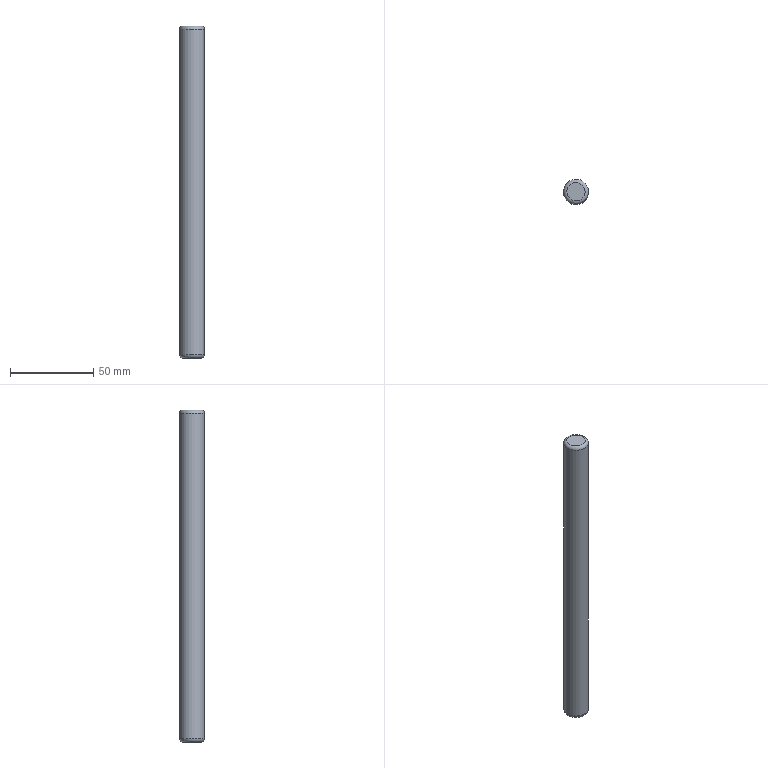Component | NX | CBK2 | 1 solid | 5 faces | box 15 x 15 x 200 mm | volume 35267 mm3 | plane 2 | torus 2 | cylinder 1 | commonest cylinder face diameters 15 x1
STEP:
#1=CARTESIAN_POINT('',(0.,0.,0.));
#2=DIRECTION('',(0.,0.,1.));
#3=DIRECTION('',(1.,0.,0.));
#4=AXIS2_PLACEMENT_3D('',#1,#2,#3);
#5=CARTESIAN_POINT('',(-1117.64,953.261,23.928));
#6=VERTEX_POINT('',#5);
#7=CARTESIAN_POINT('',(-1123.378,958.091,23.928));
#8=DIRECTION('',(0.,0.,1.));
#9=DIRECTION('',(0.7651,-0.644,0.));
#10=AXIS2_PLACEMENT_3D('',#7,#8,#9);
#11=CIRCLE('',#10,7.5);
#12=CARTESIAN_POINT('',(-1123.378,958.091,221.928));
#13=DIRECTION('',(0.,0.,-1.));
#14=DIRECTION('',(-0.7651,0.644,0.));
#15=AXIS2_PLACEMENT_3D('',#12,#13,#14);
#16=CYLINDRICAL_SURFACE('',#15,7.5);
#17=CARTESIAN_POINT('',(9.425,198.));
#18=DIRECTION('',(-1.,0.));
#19=VECTOR('',#18,1.);
#20=LINE('',#17,#19);
#21=(GEOMETRIC_REPRESENTATION_CONTEXT(2)PARAMETRIC_REPRESENTATION_CONTEXT()REPRESENTATION_CONTEXT('',''));
#22=DEFINITIONAL_REPRESENTATION('',(#20),#21);
#23=PCURVE('',#16,#22);
#24=CARTESIAN_POINT('',(-1123.378,958.091,23.928));
#25=DIRECTION('',(0.,0.,1.));
#26=DIRECTION('',(0.7651,-0.644,0.));
#27=AXIS2_PLACEMENT_3D('',#24,#25,#26);
#28=TOROIDAL_SURFACE('',#27,5.5,2.);
#29=CARTESIAN_POINT('',(0.,6.283));
#30=DIRECTION('',(1.,0.));
#31=VECTOR('',#30,1.);
#32=LINE('',#29,#31);
#33=(GEOMETRIC_REPRESENTATION_CONTEXT(2)PARAMETRIC_REPRESENTATION_CONTEXT()REPRESENTATION_CONTEXT('',''));
#34=DEFINITIONAL_REPRESENTATION('',(#32),#33);
#35=PCURVE('',#28,#34);
#36=SURFACE_CURVE('',#11,(#23,#35),.PCURVE_S1.);
#37=EDGE_CURVE('',#6,#6,#36,.T.);
#38=ORIENTED_EDGE('',*,*,#37,.T.);
#39=CARTESIAN_POINT('',(-1117.64,953.261,219.928));
#40=VERTEX_POINT('',#39);
#41=CARTESIAN_POINT('',(-1117.64,953.261,219.928));
#42=CARTESIAN_POINT('',(-1117.64,953.261,23.928));
#43=B_SPLINE_CURVE_WITH_KNOTS('',1,(#41,#42),.UNSPECIFIED.,.F.,.F.,(2,2),(2.,198.),.PIECEWISE_BEZIER_KNOTS.);
#44=CARTESIAN_POINT('',(3.142,0.));
#45=DIRECTION('',(0.,1.));
#46=VECTOR('',#45,1.);
#47=LINE('',#44,#46);
#48=(GEOMETRIC_REPRESENTATION_CONTEXT(2)PARAMETRIC_REPRESENTATION_CONTEXT()REPRESENTATION_CONTEXT('',''));
#49=DEFINITIONAL_REPRESENTATION('',(#47),#48);
#50=PCURVE('',#16,#49);
#51=CARTESIAN_POINT('',(9.425,0.));
#52=DIRECTION('',(0.,1.));
#53=VECTOR('',#52,1.);
#54=LINE('',#51,#53);
#55=(GEOMETRIC_REPRESENTATION_CONTEXT(2)PARAMETRIC_REPRESENTATION_CONTEXT()REPRESENTATION_CONTEXT('',''));
#56=DEFINITIONAL_REPRESENTATION('',(#54),#55);
#57=PCURVE('',#16,#56);
#58=SEAM_CURVE('',#43,(#50,#57),.PCURVE_S1.);
#59=EDGE_CURVE('',#40,#6,#58,.T.);
#60=ORIENTED_EDGE('',*,*,#59,.F.);
#61=CARTESIAN_POINT('',(-1123.378,958.091,219.928));
#62=DIRECTION('',(0.,0.,-1.));
#63=DIRECTION('',(0.7651,-0.644,0.));
#64=AXIS2_PLACEMENT_3D('',#61,#62,#63);
#65=CIRCLE('',#64,7.5);
#66=CARTESIAN_POINT('',(3.142,2.));
#67=DIRECTION('',(1.,0.));
#68=VECTOR('',#67,1.);
#69=LINE('',#66,#68);
#70=(GEOMETRIC_REPRESENTATION_CONTEXT(2)PARAMETRIC_REPRESENTATION_CONTEXT()REPRESENTATION_CONTEXT('',''));
#71=DEFINITIONAL_REPRESENTATION('',(#69),#70);
#72=PCURVE('',#16,#71);
#73=CARTESIAN_POINT('',(-1123.378,958.091,219.928));
#74=DIRECTION('',(0.,0.,1.));
#75=DIRECTION('',(0.7651,-0.644,0.));
#76=AXIS2_PLACEMENT_3D('',#73,#74,#75);
#77=TOROIDAL_SURFACE('',#76,5.5,2.);
#78=CARTESIAN_POINT('',(6.283,6.283));
#79=DIRECTION('',(-1.,0.));
#80=VECTOR('',#79,1.);
#81=LINE('',#78,#80);
#82=(GEOMETRIC_REPRESENTATION_CONTEXT(2)PARAMETRIC_REPRESENTATION_CONTEXT()REPRESENTATION_CONTEXT('',''));
#83=DEFINITIONAL_REPRESENTATION('',(#81),#82);
#84=PCURVE('',#77,#83);
#85=SURFACE_CURVE('',#65,(#72,#84),.PCURVE_S1.);
#86=EDGE_CURVE('',#40,#40,#85,.T.);
#87=ORIENTED_EDGE('',*,*,#86,.T.);
#88=ORIENTED_EDGE('',*,*,#59,.T.);
#89=EDGE_LOOP('',(#38,#60,#87,#88));
#90=FACE_BOUND('',#89,.T.);
#91=ADVANCED_FACE('',(#90),#16,.T.);
#92=CARTESIAN_POINT('',(-1119.171,954.549,221.928));
#93=VERTEX_POINT('',#92);
#94=CARTESIAN_POINT('',(-1123.378,958.091,221.928));
#95=DIRECTION('',(0.,0.,1.));
#96=DIRECTION('',(0.7651,-0.644,0.));
#97=AXIS2_PLACEMENT_3D('',#94,#95,#96);
#98=CIRCLE('',#97,5.5);
#99=CARTESIAN_POINT('',(-1123.378,958.091,221.928));
#100=DIRECTION('',(0.,0.,1.));
#101=DIRECTION('',(0.7651,-0.644,0.));
#102=AXIS2_PLACEMENT_3D('',#99,#100,#101);
#103=PLANE('',#102);
#104=CARTESIAN_POINT('',(0.,0.));
#105=DIRECTION('',(1.,0.));
#106=AXIS2_PLACEMENT_2D('',#104,#105);
#107=CIRCLE('',#106,5.5);
#108=(GEOMETRIC_REPRESENTATION_CONTEXT(2)PARAMETRIC_REPRESENTATION_CONTEXT()REPRESENTATION_CONTEXT('',''));
#109=DEFINITIONAL_REPRESENTATION('',(#107),#108);
#110=PCURVE('',#103,#109);
#111=CARTESIAN_POINT('',(0.,7.854));
#112=DIRECTION('',(1.,0.));
#113=VECTOR('',#112,1.);
#114=LINE('',#111,#113);
#115=(GEOMETRIC_REPRESENTATION_CONTEXT(2)PARAMETRIC_REPRESENTATION_CONTEXT()REPRESENTATION_CONTEXT('',''));
#116=DEFINITIONAL_REPRESENTATION('',(#114),#115);
#117=PCURVE('',#77,#116);
#118=SURFACE_CURVE('',#98,(#110,#117),.PCURVE_S1.);
#119=EDGE_CURVE('',#93,#93,#118,.T.);
#120=ORIENTED_EDGE('',*,*,#119,.T.);
#121=EDGE_LOOP('',(#120));
#122=FACE_BOUND('',#121,.T.);
#123=ADVANCED_FACE('',(#122),#103,.T.);
#124=CARTESIAN_POINT('',(-1119.171,954.549,21.928));
#125=VERTEX_POINT('',#124);
#126=CARTESIAN_POINT('',(-1123.378,958.091,21.928));
#127=DIRECTION('',(0.,0.,-1.));
#128=DIRECTION('',(0.7651,-0.644,0.));
#129=AXIS2_PLACEMENT_3D('',#126,#127,#128);
#130=CIRCLE('',#129,5.5);
#131=CARTESIAN_POINT('',(-1123.378,958.091,21.928));
#132=DIRECTION('',(0.,0.,1.));
#133=DIRECTION('',(0.7651,-0.644,0.));
#134=AXIS2_PLACEMENT_3D('',#131,#132,#133);
#135=PLANE('',#134);
#136=CARTESIAN_POINT('',(5.5,0.));
#137=CARTESIAN_POINT('',(5.5,-9.526));
#138=CARTESIAN_POINT('',(-2.75,-4.763));
#139=CARTESIAN_POINT('',(-11.,-0.));
#140=CARTESIAN_POINT('',(-2.75,4.763));
#141=CARTESIAN_POINT('',(5.5,9.526));
#142=CARTESIAN_POINT('',(5.5,0.));
#143=(BOUNDED_CURVE()B_SPLINE_CURVE(2,(#136,#137,#138,#139,#140,#141,#142),.UNSPECIFIED.,.T.,.F.)B_SPLINE_CURVE_WITH_KNOTS((1,2,2,2,2,1),(-2.094,0.,2.094,4.189,6.283,8.378),.UNSPECIFIED.)CURVE()GEOMETRIC_REPRESENTATION_ITEM()RATIONAL_B_SPLINE_CURVE((1.,0.5,1.,0.5,1.,0.5,1.))REPRESENTATION_ITEM(''));
#144=(GEOMETRIC_REPRESENTATION_CONTEXT(2)PARAMETRIC_REPRESENTATION_CONTEXT()REPRESENTATION_CONTEXT('',''));
#145=DEFINITIONAL_REPRESENTATION('',(#143),#144);
#146=PCURVE('',#135,#145);
#147=CARTESIAN_POINT('',(6.283,4.712));
#148=DIRECTION('',(-1.,0.));
#149=VECTOR('',#148,1.);
#150=LINE('',#147,#149);
#151=(GEOMETRIC_REPRESENTATION_CONTEXT(2)PARAMETRIC_REPRESENTATION_CONTEXT()REPRESENTATION_CONTEXT('',''));
#152=DEFINITIONAL_REPRESENTATION('',(#150),#151);
#153=PCURVE('',#28,#152);
#154=SURFACE_CURVE('',#130,(#146,#153),.PCURVE_S1.);
#155=EDGE_CURVE('',#125,#125,#154,.T.);
#156=ORIENTED_EDGE('',*,*,#155,.T.);
#157=EDGE_LOOP('',(#156));
#158=FACE_BOUND('',#157,.T.);
#159=ADVANCED_FACE('',(#158),#135,.F.);
#160=ORIENTED_EDGE('',*,*,#155,.F.);
#161=CARTESIAN_POINT('',(-1119.171,954.549,21.928));
#162=CARTESIAN_POINT('',(-1118.761,954.205,21.928));
#163=CARTESIAN_POINT('',(-1118.363,953.87,22.098));
#164=CARTESIAN_POINT('',(-1118.02,953.581,22.424));
#165=CARTESIAN_POINT('',(-1117.77,953.371,22.872));
#166=CARTESIAN_POINT('',(-1117.64,953.261,23.393));
#167=CARTESIAN_POINT('',(-1117.64,953.261,23.928));
#168=(BOUNDED_CURVE()B_SPLINE_CURVE(6,(#161,#162,#163,#164,#165,#166,#167),.UNSPECIFIED.,.F.,.F.)B_SPLINE_CURVE_WITH_KNOTS((7,7),(4.712,6.283),.PIECEWISE_BEZIER_KNOTS.)CURVE()GEOMETRIC_REPRESENTATION_ITEM()RATIONAL_B_SPLINE_CURVE((1.031,1.01,0.9979,0.994,0.9979,1.01,1.031))REPRESENTATION_ITEM(''));
#169=CARTESIAN_POINT('',(6.283,0.));
#170=DIRECTION('',(0.,1.));
#171=VECTOR('',#170,1.);
#172=LINE('',#169,#171);
#173=(GEOMETRIC_REPRESENTATION_CONTEXT(2)PARAMETRIC_REPRESENTATION_CONTEXT()REPRESENTATION_CONTEXT('',''));
#174=DEFINITIONAL_REPRESENTATION('',(#172),#173);
#175=PCURVE('',#28,#174);
#176=CARTESIAN_POINT('',(0.,0.));
#177=DIRECTION('',(0.,1.));
#178=VECTOR('',#177,1.);
#179=LINE('',#176,#178);
#180=(GEOMETRIC_REPRESENTATION_CONTEXT(2)PARAMETRIC_REPRESENTATION_CONTEXT()REPRESENTATION_CONTEXT('',''));
#181=DEFINITIONAL_REPRESENTATION('',(#179),#180);
#182=PCURVE('',#28,#181);
#183=SEAM_CURVE('',#168,(#175,#182),.PCURVE_S1.);
#184=EDGE_CURVE('',#125,#6,#183,.T.);
#185=ORIENTED_EDGE('',*,*,#184,.T.);
#186=ORIENTED_EDGE('',*,*,#37,.F.);
#187=ORIENTED_EDGE('',*,*,#184,.F.);
#188=EDGE_LOOP('',(#160,#185,#186,#187));
#189=FACE_BOUND('',#188,.T.);
#190=ADVANCED_FACE('',(#189),#28,.T.);
#191=ORIENTED_EDGE('',*,*,#86,.F.);
#192=CARTESIAN_POINT('',(-1117.64,953.261,219.928));
#193=CARTESIAN_POINT('',(-1117.64,953.261,220.462));
#194=CARTESIAN_POINT('',(-1117.77,953.371,220.983));
#195=CARTESIAN_POINT('',(-1118.02,953.581,221.431));
#196=CARTESIAN_POINT('',(-1118.363,953.87,221.757));
#197=CARTESIAN_POINT('',(-1118.761,954.205,221.928));
#198=CARTESIAN_POINT('',(-1119.171,954.549,221.928));
#199=(BOUNDED_CURVE()B_SPLINE_CURVE(6,(#192,#193,#194,#195,#196,#197,#198),.UNSPECIFIED.,.F.,.F.)B_SPLINE_CURVE_WITH_KNOTS((7,7),(0.,1.571),.PIECEWISE_BEZIER_KNOTS.)CURVE()GEOMETRIC_REPRESENTATION_ITEM()RATIONAL_B_SPLINE_CURVE((1.031,1.01,0.9979,0.994,0.9979,1.01,1.031))REPRESENTATION_ITEM(''));
#200=CARTESIAN_POINT('',(6.283,6.283));
#201=DIRECTION('',(0.,1.));
#202=VECTOR('',#201,1.);
#203=LINE('',#200,#202);
#204=(GEOMETRIC_REPRESENTATION_CONTEXT(2)PARAMETRIC_REPRESENTATION_CONTEXT()REPRESENTATION_CONTEXT('',''));
#205=DEFINITIONAL_REPRESENTATION('',(#203),#204);
#206=PCURVE('',#77,#205);
#207=CARTESIAN_POINT('',(0.,6.283));
#208=DIRECTION('',(0.,1.));
#209=VECTOR('',#208,1.);
#210=LINE('',#207,#209);
#211=(GEOMETRIC_REPRESENTATION_CONTEXT(2)PARAMETRIC_REPRESENTATION_CONTEXT()REPRESENTATION_CONTEXT('',''));
#212=DEFINITIONAL_REPRESENTATION('',(#210),#211);
#213=PCURVE('',#77,#212);
#214=SEAM_CURVE('',#199,(#206,#213),.PCURVE_S1.);
#215=EDGE_CURVE('',#40,#93,#214,.T.);
#216=ORIENTED_EDGE('',*,*,#215,.T.);
#217=ORIENTED_EDGE('',*,*,#119,.F.);
#218=ORIENTED_EDGE('',*,*,#215,.F.);
#219=EDGE_LOOP('',(#191,#216,#217,#218));
#220=FACE_BOUND('',#219,.T.);
#221=ADVANCED_FACE('',(#220),#77,.T.);
#222=CLOSED_SHELL('',(#91,#123,#159,#190,#221));
#223=MANIFOLD_SOLID_BREP('',#222);
#224=(LENGTH_UNIT()NAMED_UNIT(*)SI_UNIT(.MILLI.,.METRE.));
#225=UNCERTAINTY_MEASURE_WITH_UNIT(LENGTH_MEASURE(0.00001),#224,'','');
#226=(NAMED_UNIT(*)PLANE_ANGLE_UNIT()SI_UNIT($,.RADIAN.));
#227=(NAMED_UNIT(*)SI_UNIT($,.STERADIAN.)SOLID_ANGLE_UNIT());
#228=(GEOMETRIC_REPRESENTATION_CONTEXT(3)GLOBAL_UNCERTAINTY_ASSIGNED_CONTEXT((#225))GLOBAL_UNIT_ASSIGNED_CONTEXT((#224,#226,#227))REPRESENTATION_CONTEXT('',''));
#229=ADVANCED_BREP_SHAPE_REPRESENTATION('',(#4,#223),#228);